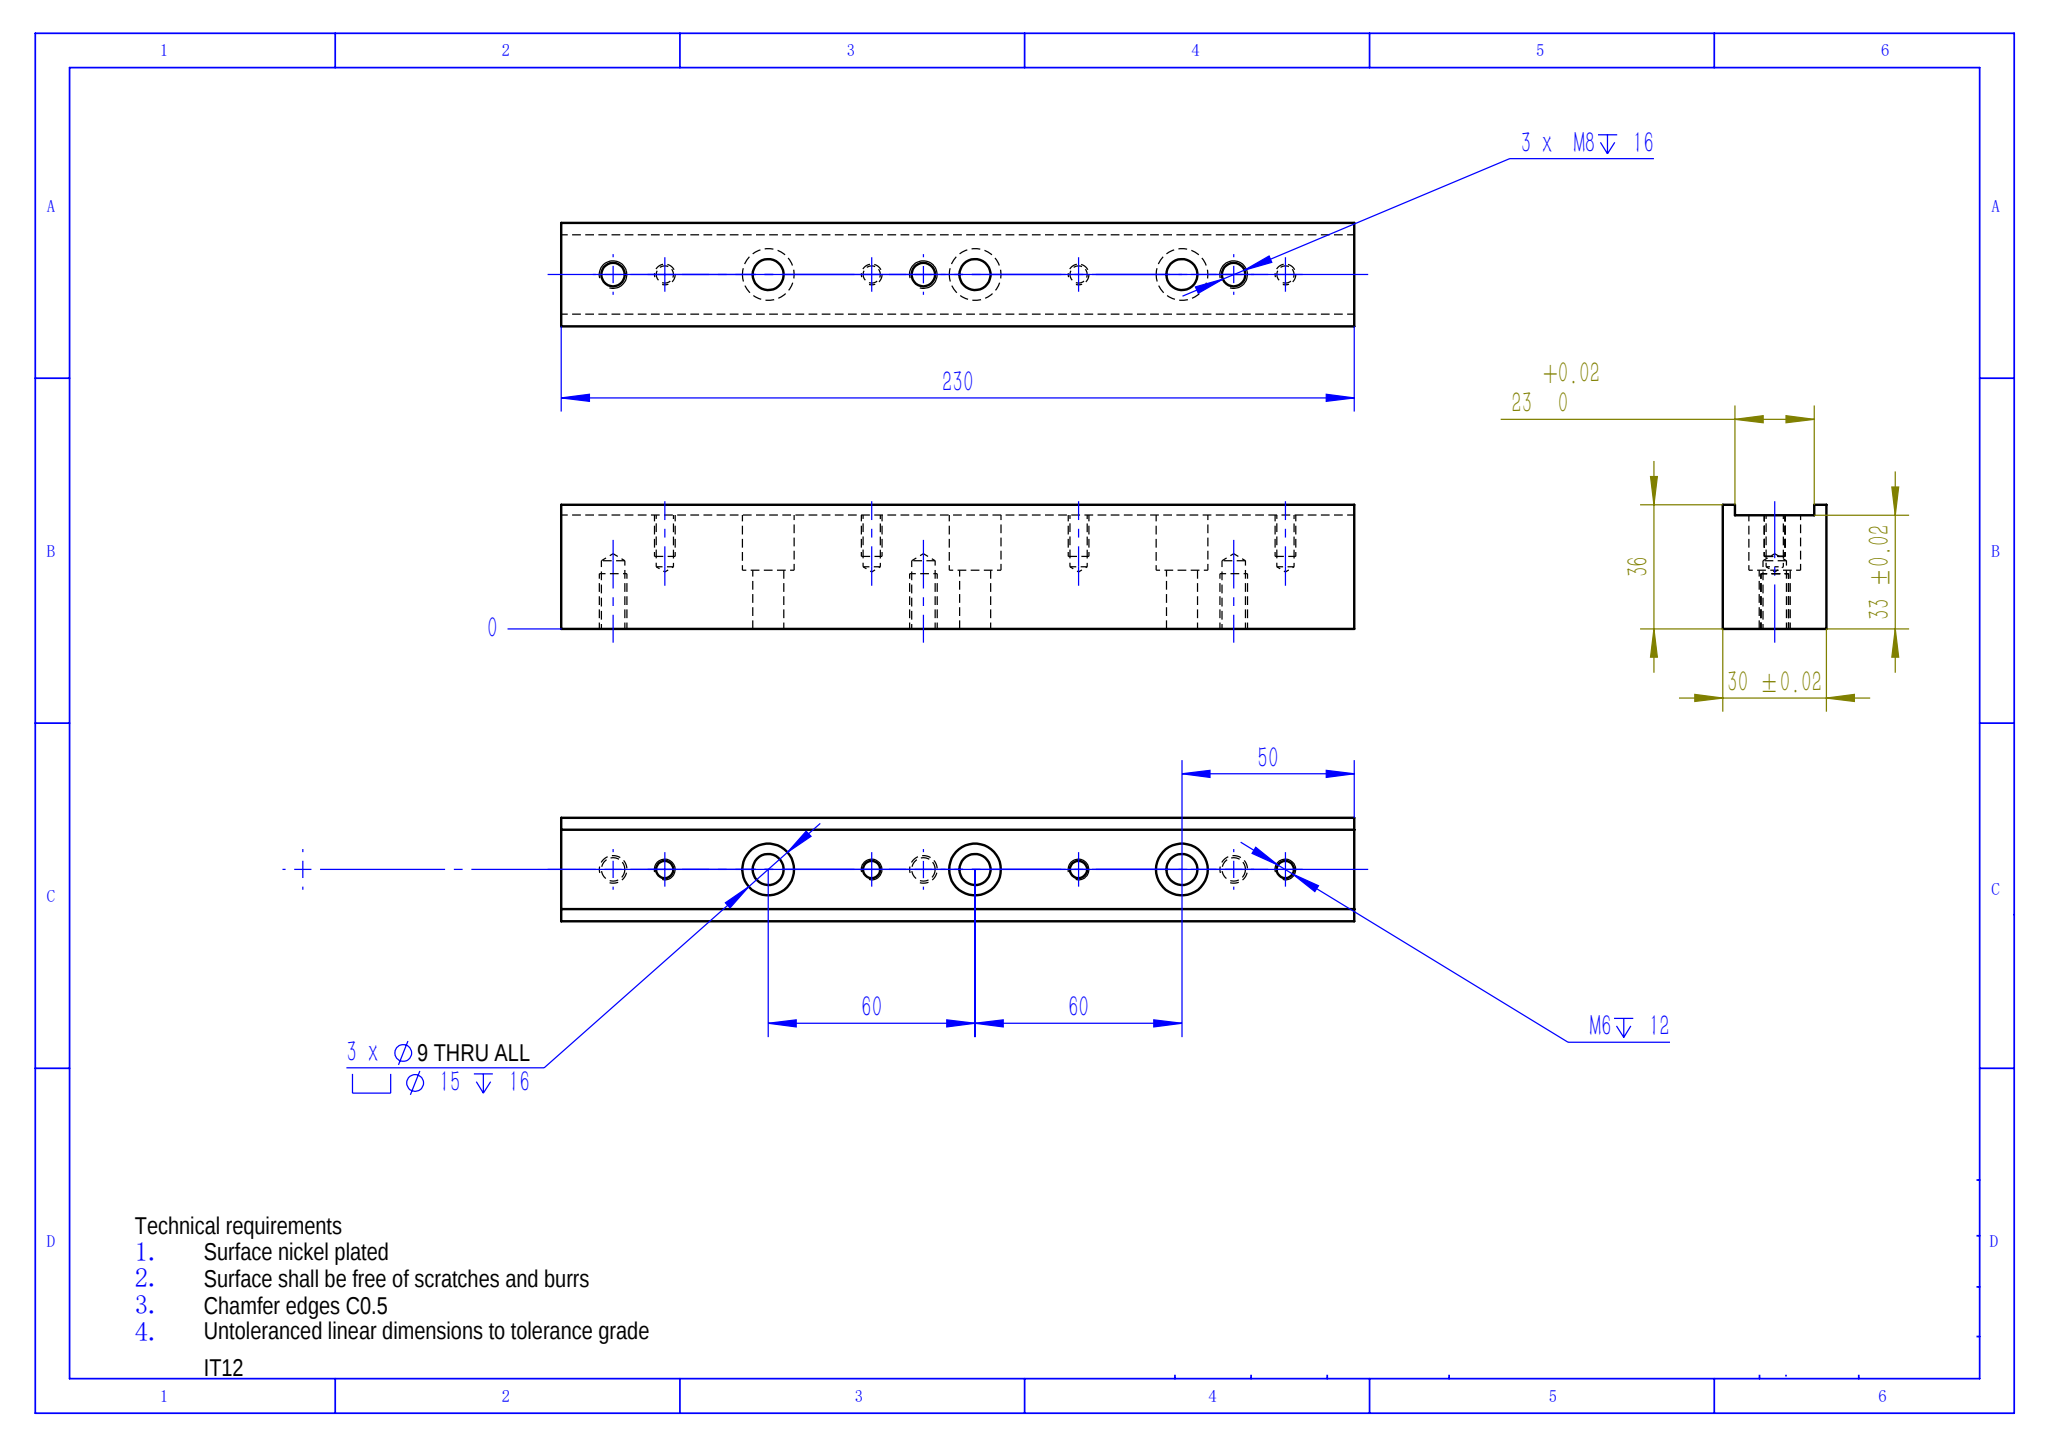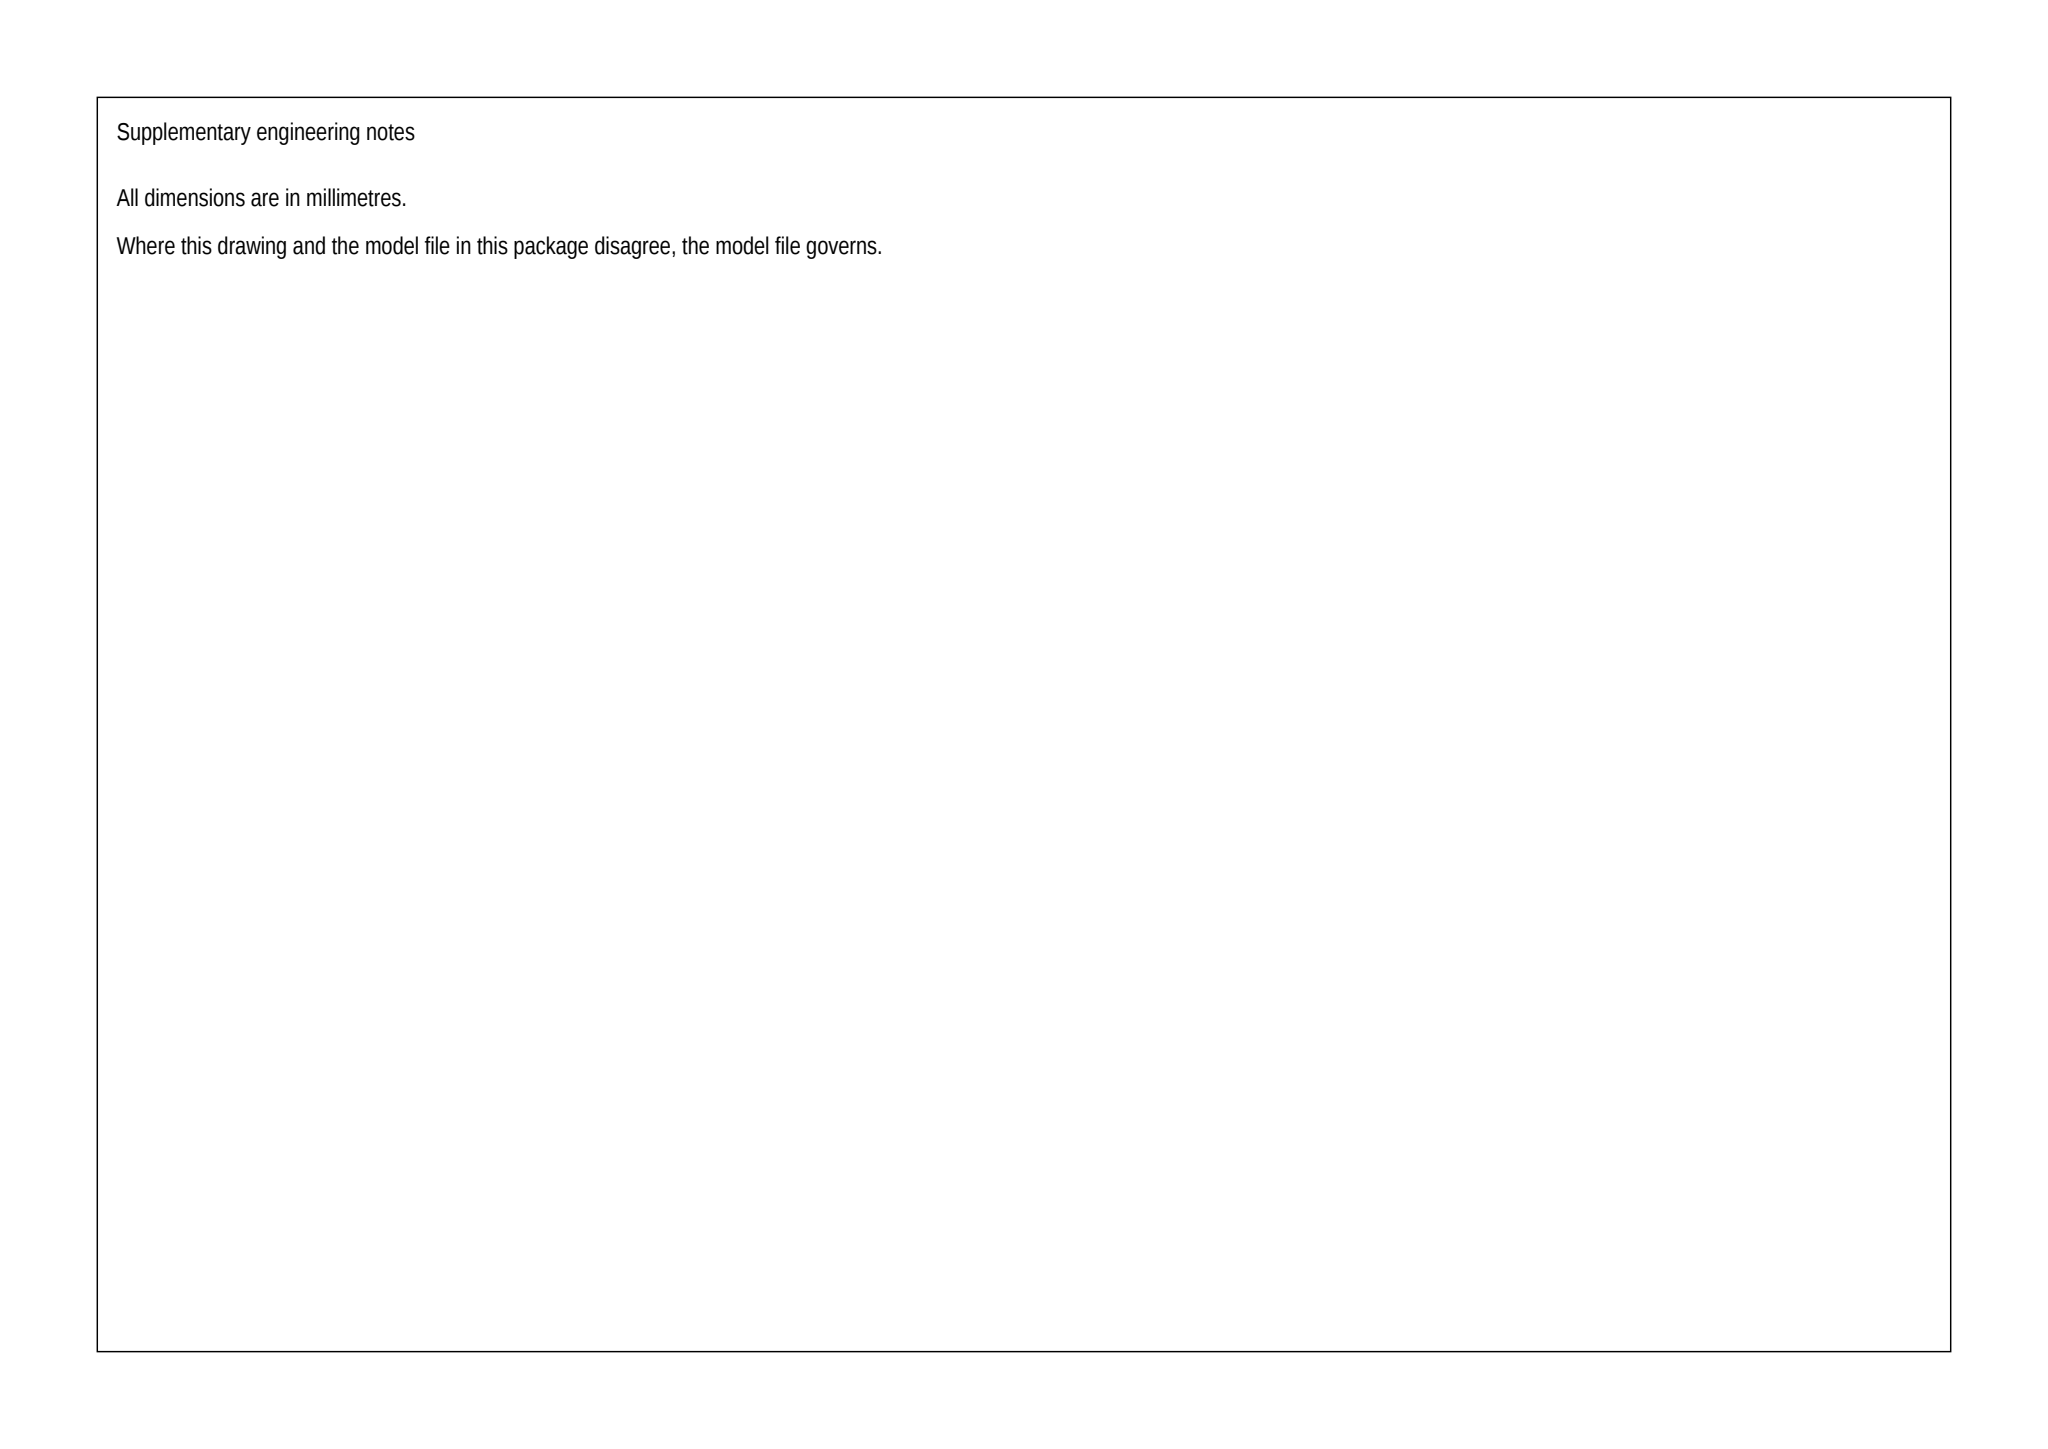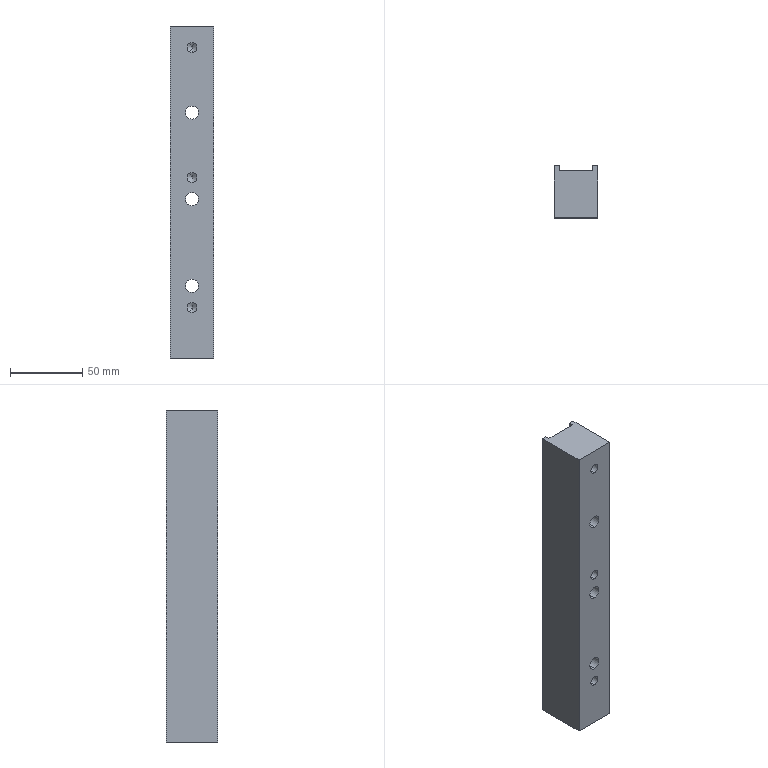Part | SolidWorks | mm | 1 solid | 53 faces | box 30 x 36 x 230 mm | volume 217360 mm3 | cylinder 26 | cone 14 | plane 13 | commonest cylinder face diameters 5 x8 15 x6 9 x6 6.8 x6
Drawing notes:
3X Ø9 THRU FROM BOTTOM FACE (Y=0), C'BORE Ø15 DP 16 FROM SLOT FLOOR (Y=33); HOLES ON PART CENTERLINE X=15, AT Z=50, 110, 170 FROM LEFT END FACE | from the solid: cylinders dia 9.0 axis y pos [15,null,50/110/170] length 17.0 and dia 15.0 axis y same positions length 16.0; axis_planes y=0, y=17, y=33
3X M8 DP 16 (TAP DRILL Ø6.8 DP 19.75), ON CENTERLINE X=15, FIRST HOLE 35 FROM LEFT END FACE (Z=0), THEN 125 AND 215 | from the solid: cylinders dia 6.8 axis y pos [15,null,35/125/215] length 19.75; cones 118° ref_dia 6.8
4X M6 DP 12 (TAP DRILL Ø5 DP 15), ON CENTERLINE X=15, AT Z=20, 80, 140, 200 FROM LEFT END FACE (Z=0) | from the solid: cylinders dia 5.0 axis y pos [15,null,20/80/140/200] length 15.0; cones 118° ref_dia 5.0
ALL DIMENSIONS IN MILLIMETERS; OVERALL SIZE 230 LONG x 30 WIDE x 36 HIGH | from the solid: bbox_xyz [30.0, 36.0, 230.0] in mm
4X M6 TAP DP 12 (TAP DRILL Ø5 DP 15), ON CENTERLINE X=15, AT Z=20, 80, 140, 200 FROM LEFT END FACE (Z=0) | from the solid: cylinders dia 5.0 axis y at [15,-,20],[15,-,80],[15,-,140],[15,-,200], length 15.0; cones 118° ref_dia 5.0
3X M8 TAP DP 16 (TAP DRILL Ø6.8 DP 19.75), ON CENTERLINE X=15, AT Z=35, 125, 215 FROM LEFT END FACE (Z=0) | from the solid: cylinders dia 6.8 axis y at [15,-,35],[15,-,125],[15,-,215], length 19.75; cones 118° ref_dia 6.8
3X Ø9 THRU FROM BOTTOM FACE (Y=0), C'BORE Ø15 DP 16 FROM SLOT FLOOR (Y=33), ON CENTERLINE X=15, AT Z=50, 110, 170 FROM LEFT END FACE (Z=0) | from the solid: cylinders dia 9.0 axis y at [15,-,50],[15,-,110],[15,-,170] length 17.0 and dia 15.0 same positions length 16.0; planes y=0, y=17, y=33
build123d program:
from build123d import *

# Parameters (mm, degrees)
BOSS_EXTRUDE1_DEPTH                               = 170
LPATTERN1_COUNT                                   = 6
LPATTERN1_PITCH                                   = 60
LPATTERN2_COUNT                                   = 4
LPATTERN2_PITCH                                   = 90
M3_TAPPED_HOLE1_D                                 = 2.5
M3_TAPPED_HOLE1_DEPTH                             = 7.5
M3_TAPPED_HOLE1_TIP                               = 0.7511
SKETCH8_W                                         = 110
SKETCH8_H                                         = 36
CUT_EXTRUDE1_DEPTH                                = 177.341
HOLE_SIZE_ACCORDING_TO_HEXAGON_SOCKET_D           = 9
HOLE_SIZE_ACCORDING_TO_HEXAGON_SOCKET_CBORE_D     = 15
HOLE_SIZE_ACCORDING_TO_HEXAGON_SOCKET_CBORE_DEPTH = 16
LPATTERN3_COUNT                                   = 3
LPATTERN3_PITCH                                   = 60


with BuildPart() as part:
    # Sketch1 → Boss-Extrude1 (new, symmetric)
    with BuildSketch(Plane.XY):
        Polygon((11.5, 36), (15, 36), (15, 0), (-15, 0), (-15, 36), (-11.5, 36), (-11.5, 33), (11.5, 33), align=None)
    extrude(amount=BOSS_EXTRUDE1_DEPTH, both=True)

    # Sketch3 → M6 Tapped Hole1 (revolve, cut)
    with BuildSketch(Plane(origin=(0, 33, 150), x_dir=(0, 0, 1), z_dir=(1, 0, 0))):
        Polygon((0, 0), (0, 16.502), (2.5, 15), (2.5, 0), align=None)
    m6_tapped_hole1 = revolve(axis=Axis((0, 39.35, 150), (0, -1, 0)), mode=Mode.SUBTRACT)

    # LPattern1: M6 Tapped Hole1 ×6
    with Locations(*[(0, 0, -i * LPATTERN1_PITCH) for i in range(1, LPATTERN1_COUNT)]):
        add(m6_tapped_hole1, mode=Mode.SUBTRACT)

    # Sketch5 → M8 Tapped Hole1 (revolve, cut)
    with BuildSketch(Plane(origin=(0, 0, -135), x_dir=(0, 0, -1), z_dir=(1, 0, 0))):
        Polygon((0, 0), (0, 21.793), (3.4, 19.75), (3.4, 0), align=None)
    m8_tapped_hole1 = revolve(axis=Axis((0, -6.35, -135), (0, 1, 0)), mode=Mode.SUBTRACT)

    # LPattern2: M8 Tapped Hole1 ×4
    with Locations(*[(0, 0, i * LPATTERN2_PITCH) for i in range(1, LPATTERN2_COUNT)]):
        add(m8_tapped_hole1, mode=Mode.SUBTRACT)

    # M3 Tapped Hole1
    with Locations(Plane(origin=(15, 0, 0), x_dir=(0, 0, -1), z_dir=(1, 0, 0))):
        with Locations((-125, 15), (-106, 15)):
            Hole(M3_TAPPED_HOLE1_D / 2, depth=M3_TAPPED_HOLE1_DEPTH)
            with Locations((0, 0, -(M3_TAPPED_HOLE1_DEPTH + M3_TAPPED_HOLE1_TIP / 2))):  # 118° drill point
                Cone(0, M3_TAPPED_HOLE1_D / 2, M3_TAPPED_HOLE1_TIP, mode=Mode.SUBTRACT)

    # Sketch8 → Cut-Extrude1 (cut, through all)
    with BuildSketch(Plane(origin=(15, 0, 0), x_dir=(0, 0, -1), z_dir=(1, 0, 0))):
        with Locations((-115, 18)):
            Rectangle(SKETCH8_W, SKETCH8_H)
    extrude(amount=-CUT_EXTRUDE1_DEPTH, mode=Mode.SUBTRACT)

    # Hole Size _ according to_ Hexagon Socket (through all)
    with Locations(Plane(origin=(0, 33, -120), x_dir=(0, 0, 1), z_dir=(0, 1, 0))):
        with Locations((0, 0)):
            hole_size_according_to_hexagon_socket = CounterBoreHole(HOLE_SIZE_ACCORDING_TO_HEXAGON_SOCKET_D / 2, HOLE_SIZE_ACCORDING_TO_HEXAGON_SOCKET_CBORE_D / 2, HOLE_SIZE_ACCORDING_TO_HEXAGON_SOCKET_CBORE_DEPTH)

    # LPattern3: Hole Size _ according to_ Hexagon Socket ×3
    with Locations(*[(0, 0, i * LPATTERN3_PITCH) for i in range(1, LPATTERN3_COUNT)]):
        add(hole_size_according_to_hexagon_socket, mode=Mode.SUBTRACT)


solid = part.part